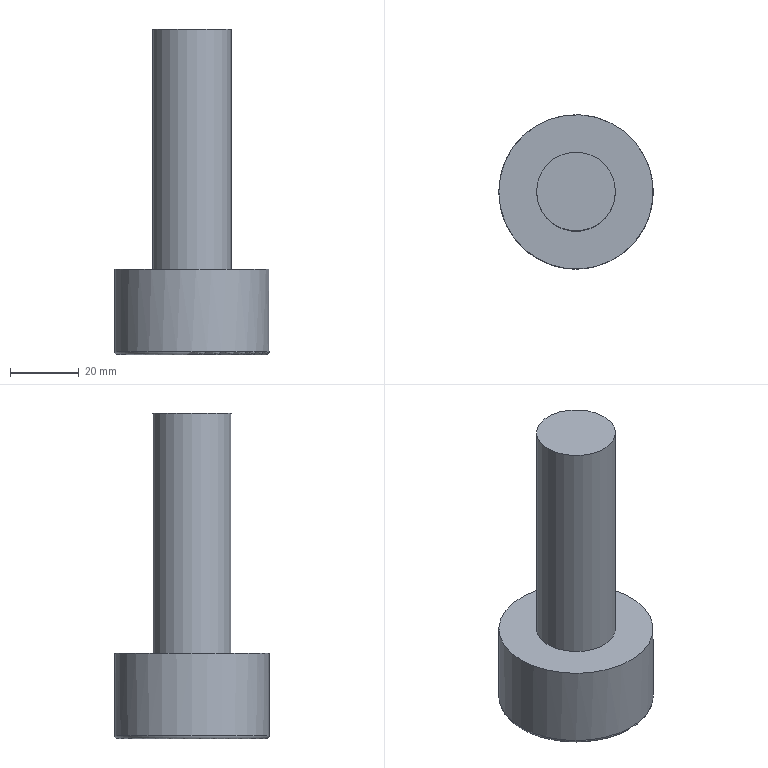Component | NX | FLANGE_TRANSITION_BOLT | 1 solid | 25 faces | volume 66380 mm3 | plane 16 | cylinder 8 | torus 1 | commonest cylinder face diameters 8 x6 45 x1 23 x1